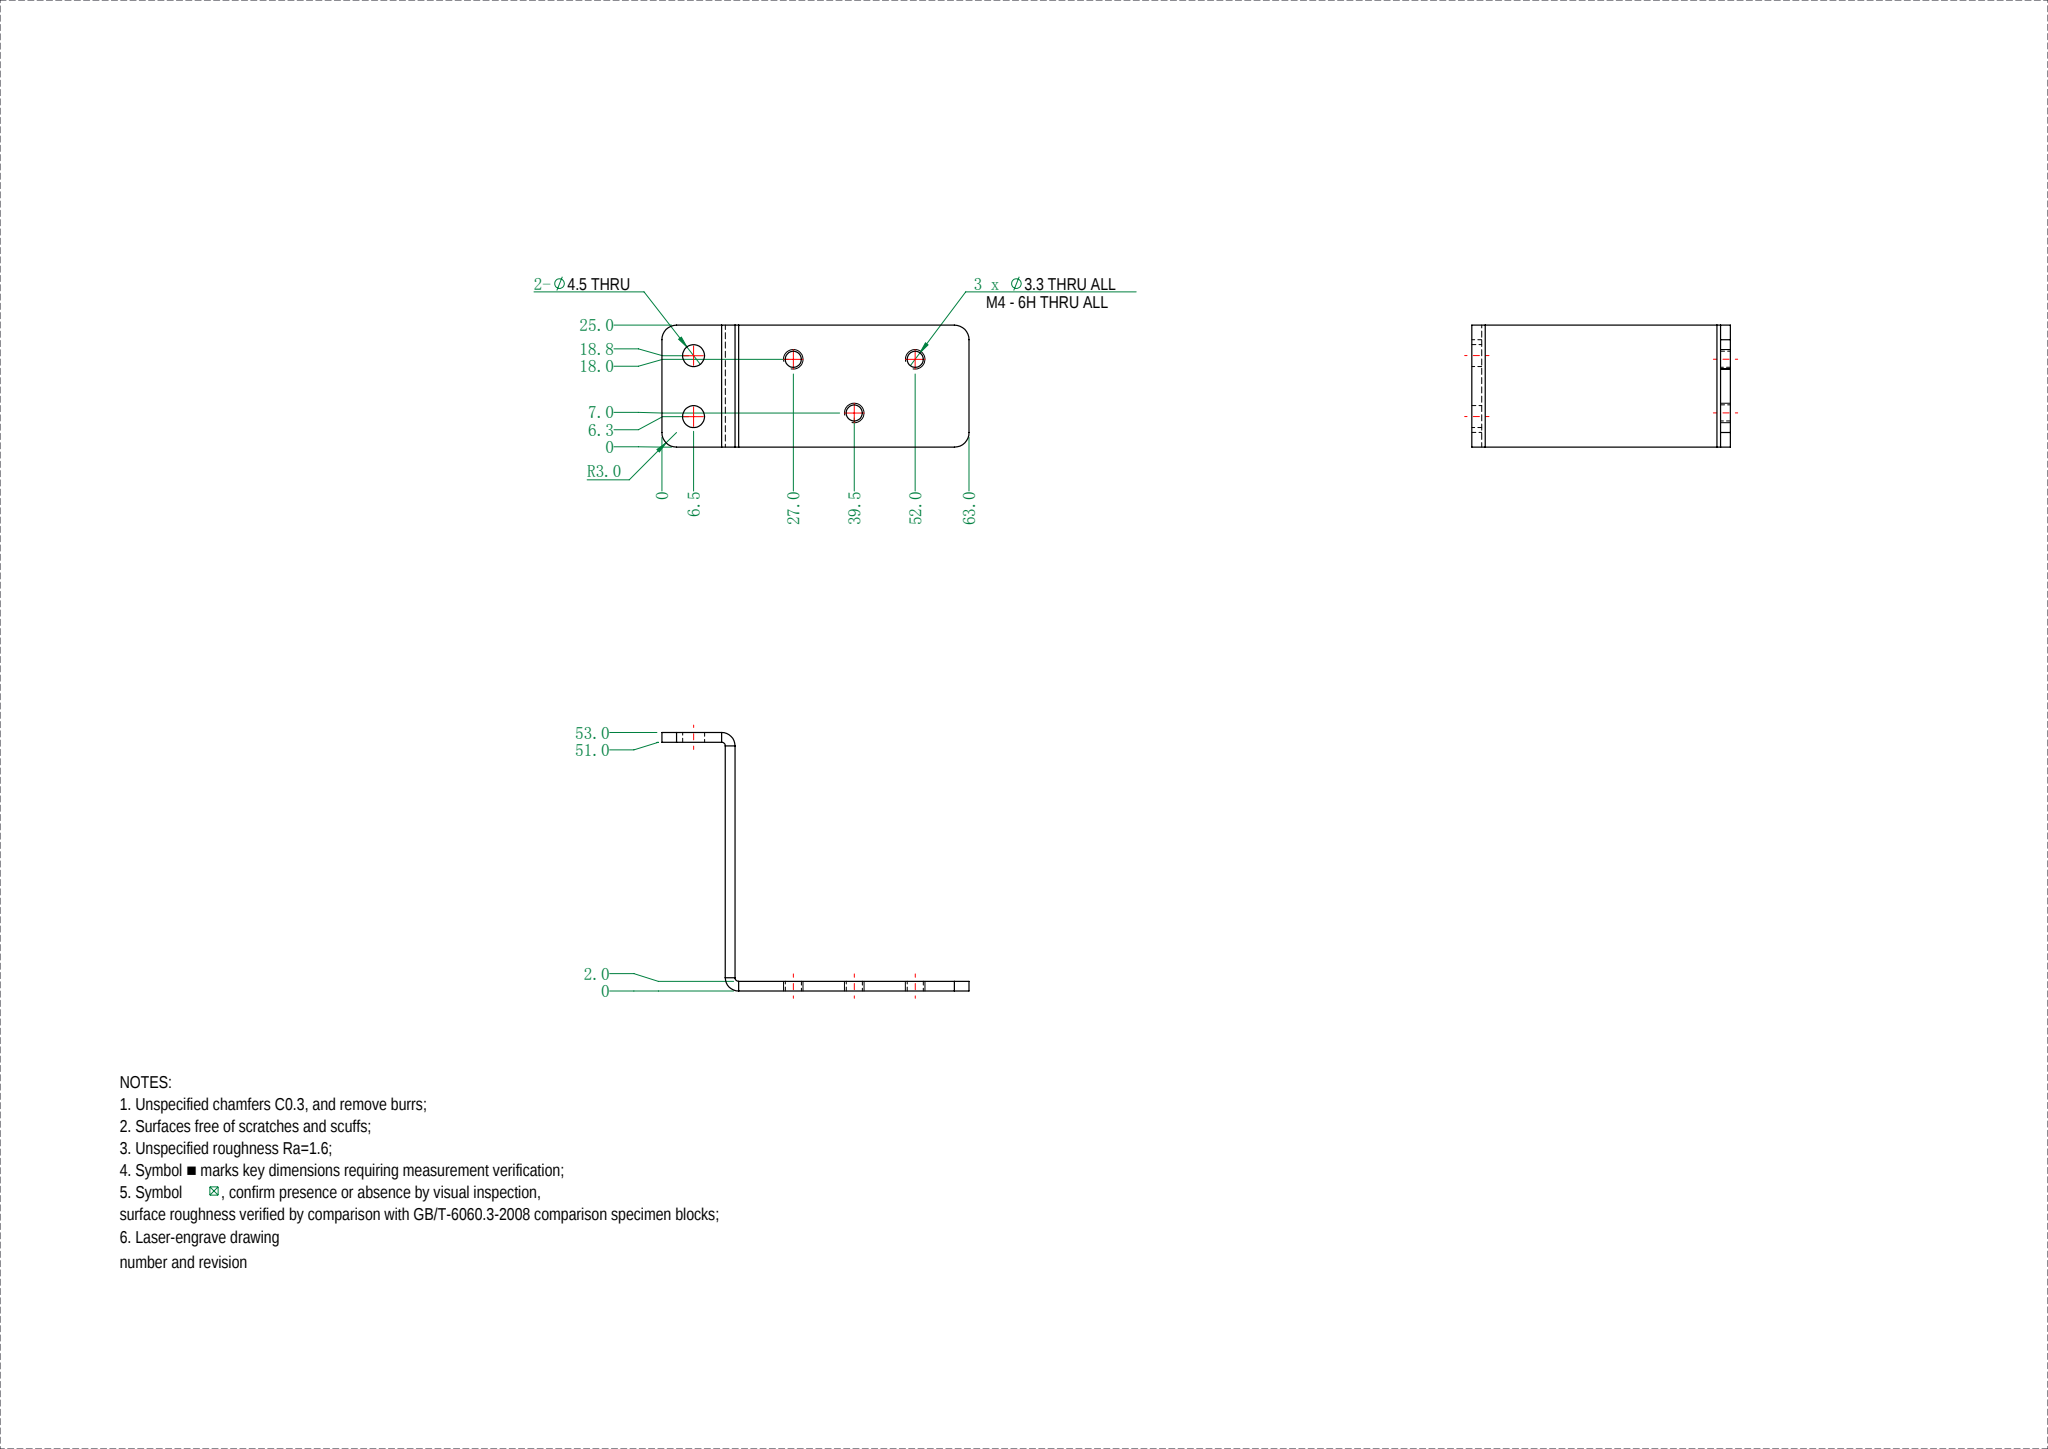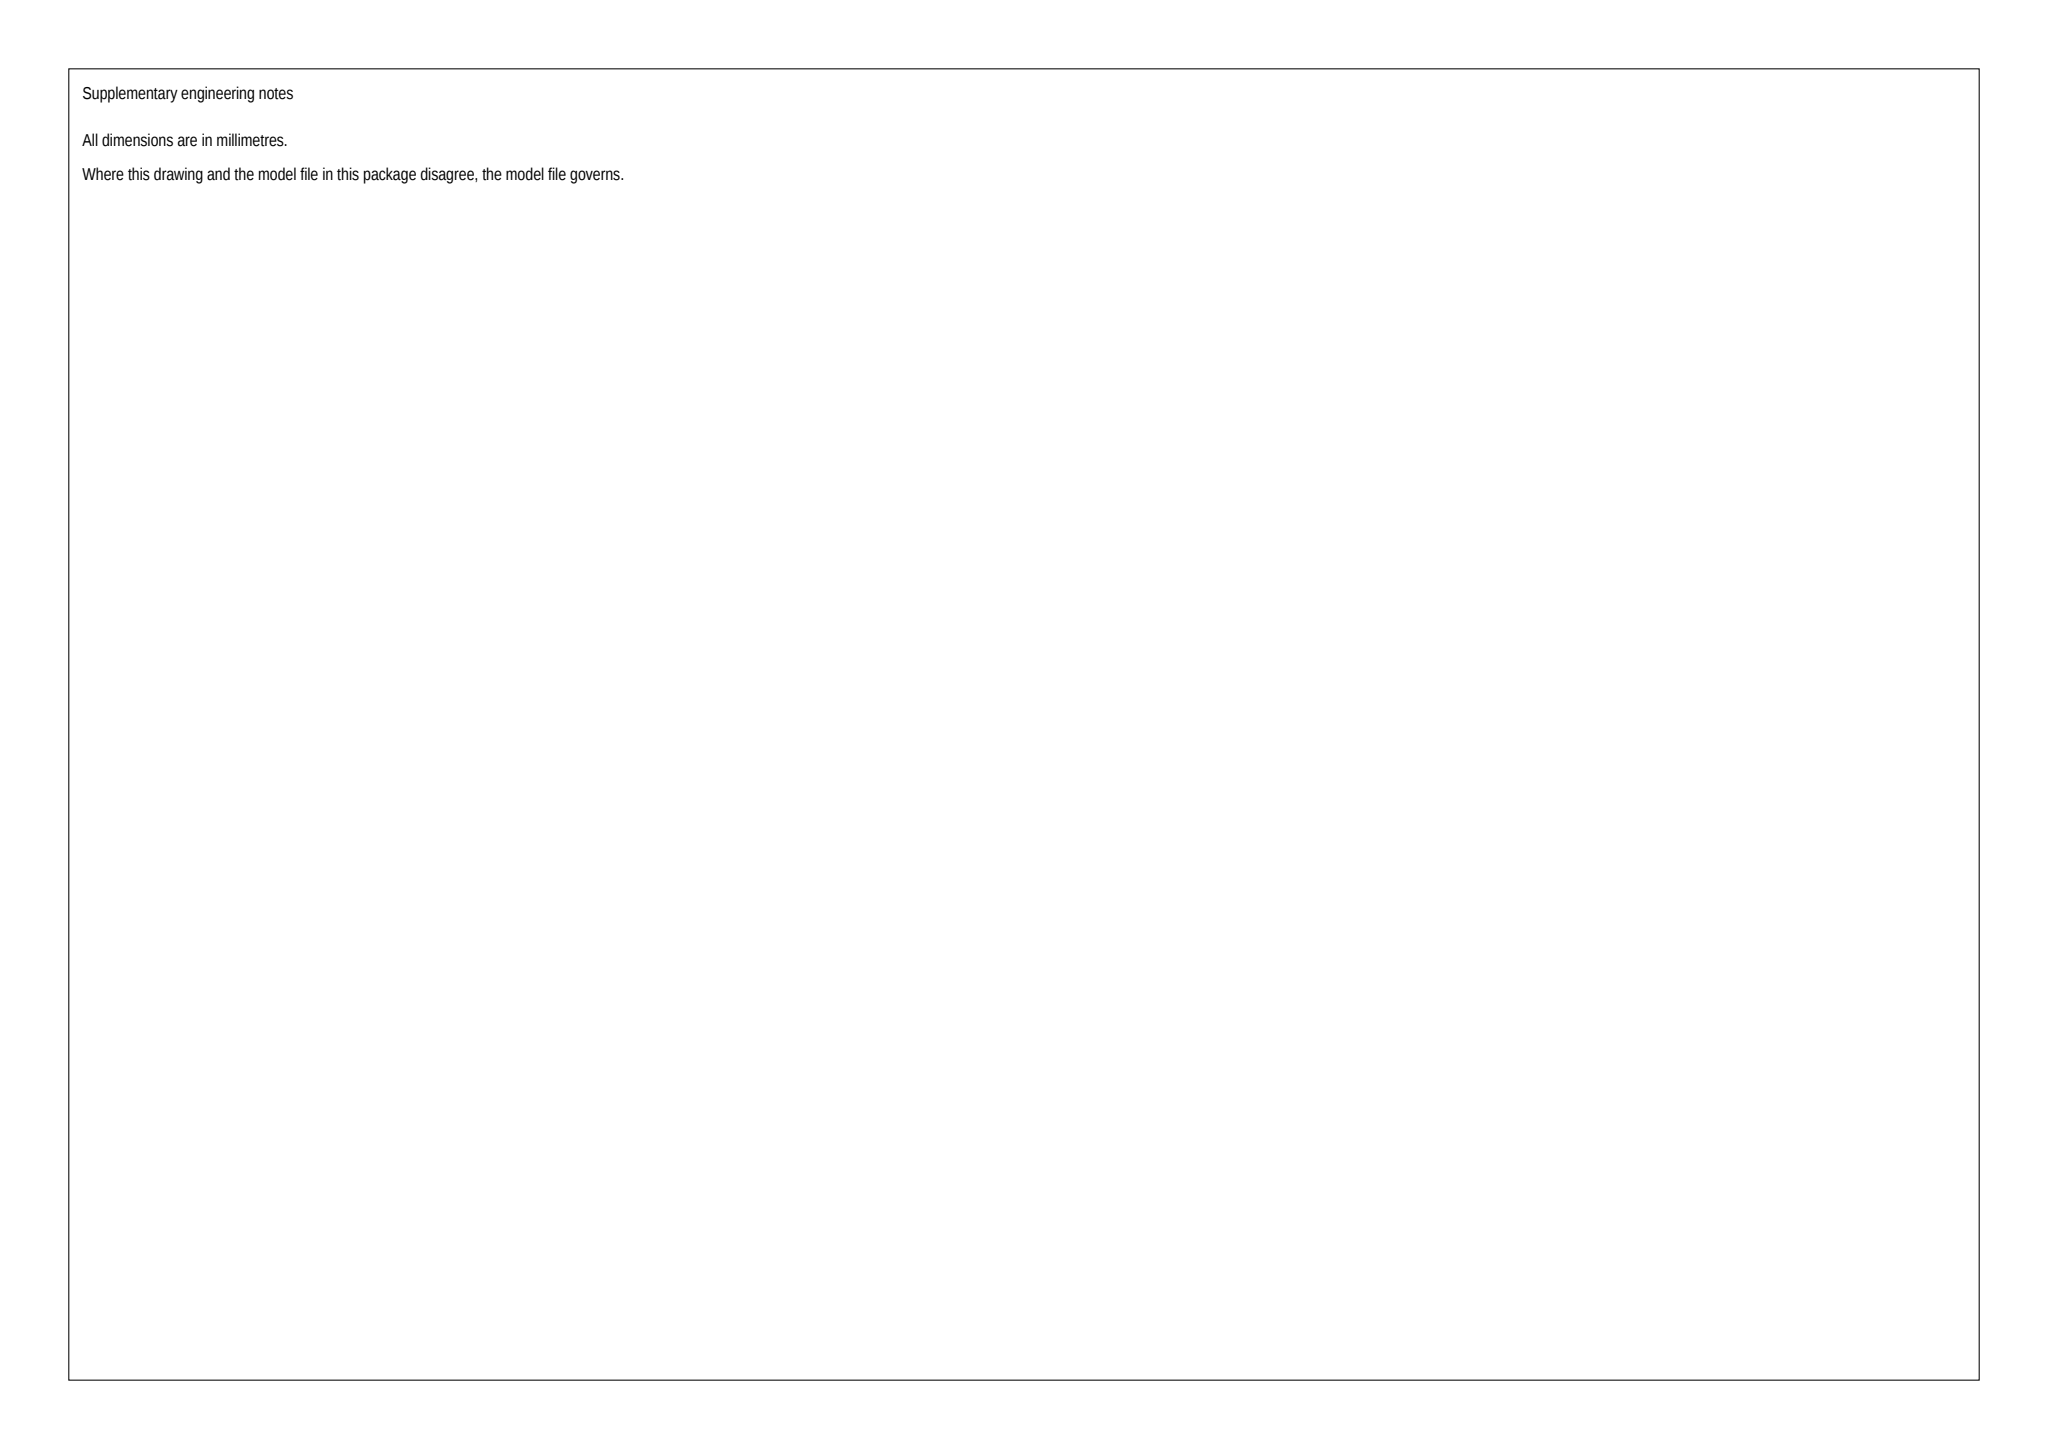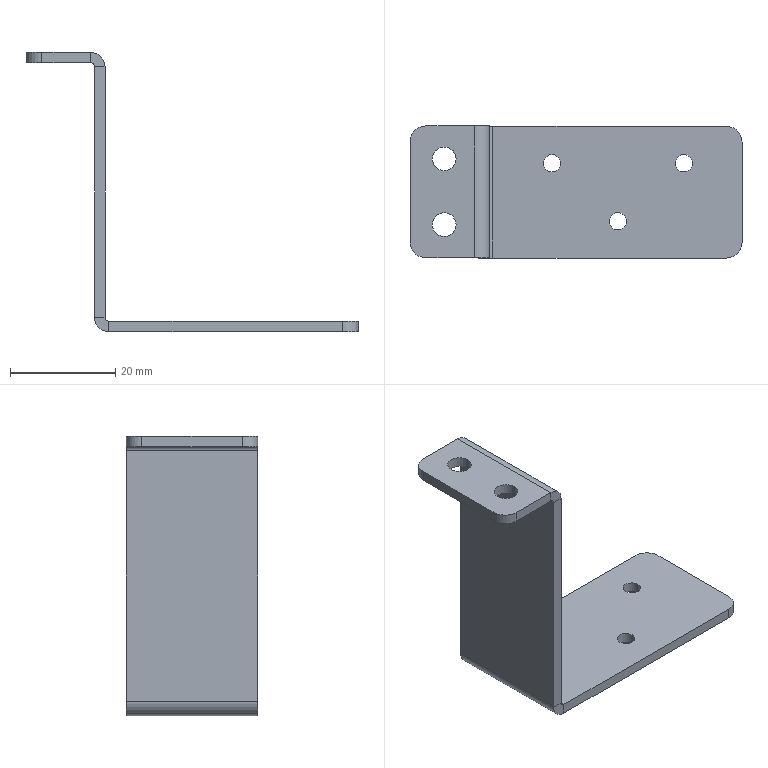Part | SolidWorks | mm | 1 solid | 36 faces | box 63 x 25 x 53 mm | volume 5495 mm3 | cylinder 18 | plane 18 | commonest cylinder face diameters 3.3 x6 4.5 x4 6 x4 5.473 x2 1.473 x2
Drawing notes:
SIDE VIEW: TOP FLANGE-TO-WEB BEND R0.7 INR / R2.74 OUTR | from the solid: Y-axis cyls at (x12.26,z50.26): dia 1.473 (R0.74) inner, dia 5.473 (R2.74) outer
SIDE VIEW: WEB 2.0 THK; FAR FACE 15.0 FROM LEFT EDGE (X0) | from the solid: x-normal planes at 13.0 and 15.0 vs datum x=0.0 (bbox X 63.0)